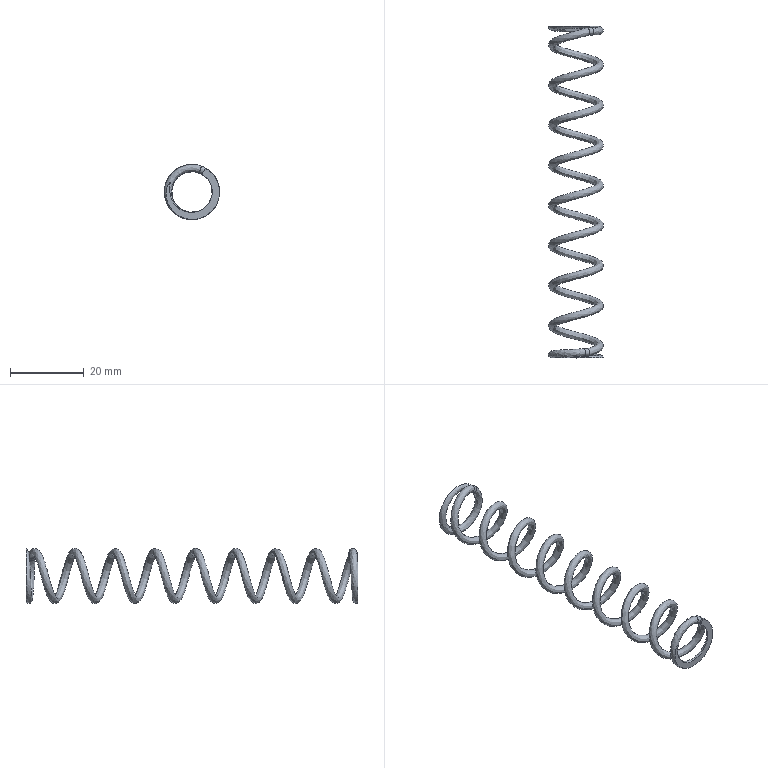Component | NX | SPRING | 1 solid | 9 faces | volume 1204 mm3 | spline 5 | plane 4